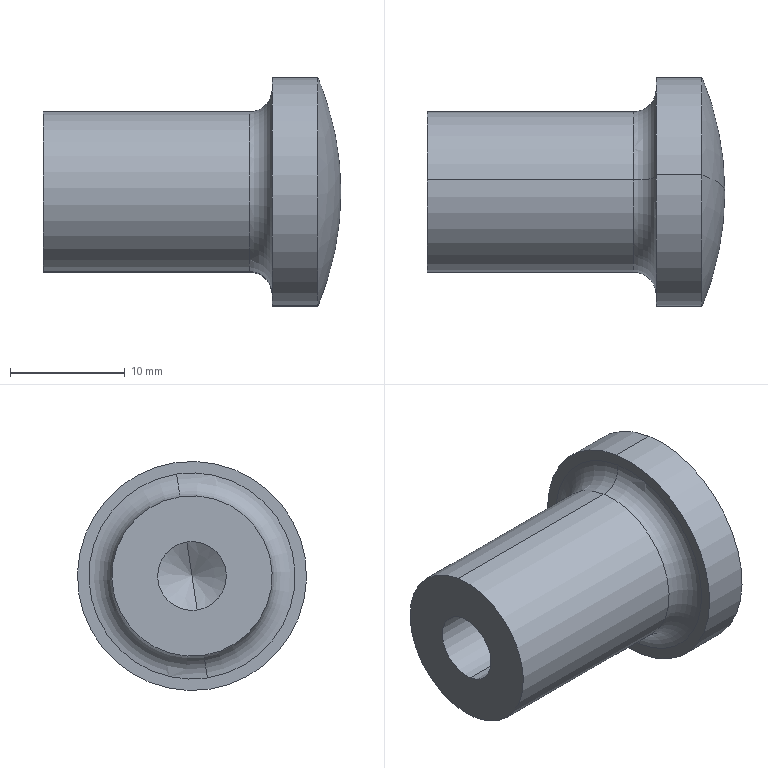Component | SolidWorks | STB-08-000-3-1_STB-08-027-1 | 1 solid | 14 faces | box 26 x 20 x 20 mm | volume 4196 mm3 | cylinder 6 | cone 2 | torus 2 | sphere 2 | plane 2 | commonest cylinder face diameters 6 x2 14 x2 20 x2
build123d program:
from build123d import *

# Parameters (mm, degrees)
SKETCH1_R             = 10
BOSS_EXTRUDE1_DEPTH   = 12
SKETCH2_OUTSIDE_W     = 29.418
SKETCH2_OUTSIDE_H     = 29.418
SKETCH2_OUTSIDE_R     = 7
CUT_EXTRUDE1_DEPTH    = 20
FILLET1_R             = 2
M6_TAPPED_HOLE1_D     = 6
M6_TAPPED_HOLE1_DEPTH = 17
M6_TAPPED_HOLE1_TIP   = 1.803
DOME1_FACE_RADIUS     = 10
DOME1_HEIGHT          = 2


with BuildPart() as part:
    # Sketch1 → Boss-Extrude1 (new, symmetric)
    with BuildSketch(Plane(origin=(0, 0, 0), x_dir=(0, 0, -1), z_dir=(1, 0, 0))):
        Circle(SKETCH1_R)
    extrude(amount=BOSS_EXTRUDE1_DEPTH, both=True)

    # Sketch2 outside → Cut-Extrude1 (cut)
    with BuildSketch(Plane.ZY.offset(12)):
        Rectangle(SKETCH2_OUTSIDE_W, SKETCH2_OUTSIDE_H)
        Circle(SKETCH2_OUTSIDE_R, mode=Mode.SUBTRACT)
    extrude(amount=-CUT_EXTRUDE1_DEPTH, mode=Mode.SUBTRACT)

    # Fillet1
    fillet1_edges = [part.edges().sort_by_distance(p)[0] for p in [
        (8, 0, -7),
    ]]
    fillet(fillet1_edges, radius=FILLET1_R)

    # M6 Tapped Hole1
    with Locations(Plane.ZY.offset(12)):
        with Locations((0, 0)):
            Hole(M6_TAPPED_HOLE1_D / 2, depth=M6_TAPPED_HOLE1_DEPTH)
            with Locations((0, 0, -(M6_TAPPED_HOLE1_DEPTH + M6_TAPPED_HOLE1_TIP / 2))):  # 118° drill point
                Cone(0, M6_TAPPED_HOLE1_D / 2, M6_TAPPED_HOLE1_TIP, mode=Mode.SUBTRACT)

    # Dome1: a dome of height H over a round flat face of radius A is a cap of a sphere of radius (A * A + H * H) / (2 * H)
    dome1_r = (DOME1_FACE_RADIUS * DOME1_FACE_RADIUS + DOME1_HEIGHT * DOME1_HEIGHT) / (2 * DOME1_HEIGHT)
    dome1_base = Plane((12, 0, 0), z_dir=(1, 0, 0))
    with Locations(dome1_base.offset(DOME1_HEIGHT - dome1_r)):
        dome1_ball = Sphere(dome1_r, mode=Mode.PRIVATE)
    add(split(dome1_ball, bisect_by=dome1_base, keep=Keep.TOP, mode=Mode.PRIVATE))


solid = part.part

# Placed as in the assembly
solid = solid.moved(Location((-207.904, 437.999, -10), (0, 0, 0)))
STEP:
#1=CARTESIAN_POINT('',(-7.988,17.226,-0.5105));
#2=VERTEX_POINT('',#1);
#3=CARTESIAN_POINT('',(-7.988,17.262,-0.2769));
#4=VERTEX_POINT('',#3);
#5=CARTESIAN_POINT('',(-7.988,17.244,-0.3937));
#6=DIRECTION('',(-1.,0.,0.));
#7=DIRECTION('',(0.,0.1487,0.9889));
#8=AXIS2_PLACEMENT_3D('',#5,#6,#7);
#9=CIRCLE('',#8,0.1181);
#10=EDGE_CURVE('',#2,#4,#9,.T.);
#11=ORIENTED_EDGE('',*,*,#10,.F.);
#12=CARTESIAN_POINT('',(-8.658,17.226,-0.5105));
#13=VERTEX_POINT('',#12);
#14=CARTESIAN_POINT('',(-8.658,17.226,-0.5105));
#15=DIRECTION('',(-1.,0.,0.));
#16=VECTOR('',#15,39.37);
#17=LINE('',#14,#16);
#18=EDGE_CURVE('',#2,#13,#17,.T.);
#19=ORIENTED_EDGE('',*,*,#18,.T.);
#20=CARTESIAN_POINT('',(-8.658,17.262,-0.2769));
#21=VERTEX_POINT('',#20);
#22=CARTESIAN_POINT('',(-8.658,17.244,-0.3937));
#23=DIRECTION('',(-1.,0.,0.));
#24=DIRECTION('',(0.,0.1487,0.9889));
#25=AXIS2_PLACEMENT_3D('',#22,#23,#24);
#26=CIRCLE('',#25,0.1181);
#27=EDGE_CURVE('',#13,#21,#26,.T.);
#28=ORIENTED_EDGE('',*,*,#27,.T.);
#29=CARTESIAN_POINT('',(-8.658,17.262,-0.2769));
#30=DIRECTION('',(-1.,0.,0.));
#31=VECTOR('',#30,39.37);
#32=LINE('',#29,#31);
#33=EDGE_CURVE('',#4,#21,#32,.T.);
#34=ORIENTED_EDGE('',*,*,#33,.F.);
#35=EDGE_LOOP('',(#11,#19,#28,#34));
#36=FACE_OUTER_BOUND('',#35,.T.);
#37=CARTESIAN_POINT('',(-8.658,17.244,-0.3937));
#38=DIRECTION('',(-1.,0.,0.));
#39=DIRECTION('',(0.,0.1487,0.9889));
#40=AXIS2_PLACEMENT_3D('',#37,#38,#39);
#41=CYLINDRICAL_SURFACE('',#40,0.1181);
#42=ADVANCED_FACE('',(#36),#41,.F.);
#43=CARTESIAN_POINT('',(-7.917,17.244,-0.3937));
#44=VERTEX_POINT('',#43);
#45=CARTESIAN_POINT('',(-7.988,17.262,-0.2769));
#46=DIRECTION('',(-0.515,0.1274,0.8476));
#47=VECTOR('',#46,39.37);
#48=LINE('',#45,#47);
#49=EDGE_CURVE('',#44,#4,#48,.T.);
#50=ORIENTED_EDGE('',*,*,#49,.F.);
#51=CARTESIAN_POINT('',(-7.988,17.226,-0.5105));
#52=DIRECTION('',(-0.515,-0.1274,-0.8476));
#53=VECTOR('',#52,39.37);
#54=LINE('',#51,#53);
#55=EDGE_CURVE('',#44,#2,#54,.T.);
#56=ORIENTED_EDGE('',*,*,#55,.T.);
#57=ORIENTED_EDGE('',*,*,#10,.T.);
#58=EDGE_LOOP('',(#50,#56,#57));
#59=FACE_OUTER_BOUND('',#58,.T.);
#60=CARTESIAN_POINT('',(-7.988,17.244,-0.3937));
#61=DIRECTION('',(-1.,0.,0.));
#62=DIRECTION('',(0.,0.1487,0.9889));
#63=AXIS2_PLACEMENT_3D('',#60,#61,#62);
#64=CONICAL_SURFACE('',#63,0.1181,1.03);
#65=ADVANCED_FACE('',(#59),#64,.F.);
#66=CARTESIAN_POINT('',(-7.949,17.203,-0.6662));
#67=VERTEX_POINT('',#66);
#68=CARTESIAN_POINT('',(-7.949,17.285,-0.1212));
#69=VERTEX_POINT('',#68);
#70=CARTESIAN_POINT('',(-7.949,17.244,-0.3937));
#71=DIRECTION('',(-1.,0.,0.));
#72=DIRECTION('',(0.,0.1487,0.9889));
#73=AXIS2_PLACEMENT_3D('',#70,#71,#72);
#74=CIRCLE('',#73,0.2756);
#75=EDGE_CURVE('',#67,#69,#74,.T.);
#76=ORIENTED_EDGE('',*,*,#75,.F.);
#77=CARTESIAN_POINT('',(-7.87,17.191,-0.7441));
#78=VERTEX_POINT('',#77);
#79=CARTESIAN_POINT('',(-7.949,17.191,-0.7441));
#80=DIRECTION('',(0.,0.9889,-0.1487));
#81=DIRECTION('',(0.,0.1487,0.9889));
#82=AXIS2_PLACEMENT_3D('',#79,#80,#81);
#83=CIRCLE('',#82,0.07874);
#84=EDGE_CURVE('',#67,#78,#83,.T.);
#85=ORIENTED_EDGE('',*,*,#84,.T.);
#86=CARTESIAN_POINT('',(-7.87,17.297,-0.04331));
#87=VERTEX_POINT('',#86);
#88=CARTESIAN_POINT('',(-7.87,17.244,-0.3937));
#89=DIRECTION('',(1.,0.,0.));
#90=DIRECTION('',(0.,0.1487,0.9889));
#91=AXIS2_PLACEMENT_3D('',#88,#89,#90);
#92=CIRCLE('',#91,0.3543);
#93=EDGE_CURVE('',#87,#78,#92,.T.);
#94=ORIENTED_EDGE('',*,*,#93,.F.);
#95=CARTESIAN_POINT('',(-7.949,17.297,-0.04331));
#96=DIRECTION('',(0.,-0.9889,0.1487));
#97=DIRECTION('',(0.,-0.1487,-0.9889));
#98=AXIS2_PLACEMENT_3D('',#95,#96,#97);
#99=CIRCLE('',#98,0.07874);
#100=EDGE_CURVE('',#69,#87,#99,.T.);
#101=ORIENTED_EDGE('',*,*,#100,.F.);
#102=EDGE_LOOP('',(#76,#85,#94,#101));
#103=FACE_OUTER_BOUND('',#102,.T.);
#104=CARTESIAN_POINT('',(-7.949,17.244,-0.3937));
#105=DIRECTION('',(-1.,0.,0.));
#106=DIRECTION('',(0.,0.1487,0.9889));
#107=AXIS2_PLACEMENT_3D('',#104,#105,#106);
#108=TOROIDAL_SURFACE('',#107,0.3543,0.07874);
#109=ADVANCED_FACE('',(#103),#108,.F.);
#110=CARTESIAN_POINT('',(-7.949,17.244,-0.3937));
#111=DIRECTION('',(-1.,0.,0.));
#112=DIRECTION('',(0.,0.1487,0.9889));
#113=AXIS2_PLACEMENT_3D('',#110,#111,#112);
#114=CIRCLE('',#113,0.2756);
#115=EDGE_CURVE('',#69,#67,#114,.T.);
#116=ORIENTED_EDGE('',*,*,#115,.T.);
#117=CARTESIAN_POINT('',(-8.658,17.203,-0.6662));
#118=VERTEX_POINT('',#117);
#119=CARTESIAN_POINT('',(-7.87,17.203,-0.6662));
#120=DIRECTION('',(-1.,0.,0.));
#121=VECTOR('',#120,39.37);
#122=LINE('',#119,#121);
#123=EDGE_CURVE('',#67,#118,#122,.T.);
#124=ORIENTED_EDGE('',*,*,#123,.T.);
#125=CARTESIAN_POINT('',(-8.658,17.285,-0.1212));
#126=VERTEX_POINT('',#125);
#127=CARTESIAN_POINT('',(-8.658,17.244,-0.3937));
#128=DIRECTION('',(-1.,0.,0.));
#129=DIRECTION('',(0.,0.1487,0.9889));
#130=AXIS2_PLACEMENT_3D('',#127,#128,#129);
#131=CIRCLE('',#130,0.2756);
#132=EDGE_CURVE('',#126,#118,#131,.T.);
#133=ORIENTED_EDGE('',*,*,#132,.F.);
#134=CARTESIAN_POINT('',(-7.87,17.285,-0.1212));
#135=DIRECTION('',(-1.,0.,0.));
#136=VECTOR('',#135,39.37);
#137=LINE('',#134,#136);
#138=EDGE_CURVE('',#69,#126,#137,.T.);
#139=ORIENTED_EDGE('',*,*,#138,.F.);
#140=EDGE_LOOP('',(#116,#124,#133,#139));
#141=FACE_OUTER_BOUND('',#140,.T.);
#142=CARTESIAN_POINT('',(-7.87,17.244,-0.3937));
#143=DIRECTION('',(-1.,0.,0.));
#144=DIRECTION('',(0.,0.1487,0.9889));
#145=AXIS2_PLACEMENT_3D('',#142,#143,#144);
#146=CYLINDRICAL_SURFACE('',#145,0.2756);
#147=ADVANCED_FACE('',(#141),#146,.T.);
#148=CARTESIAN_POINT('',(-7.713,17.303,-0.004375));
#149=VERTEX_POINT('',#148);
#150=CARTESIAN_POINT('',(-7.713,17.186,-0.783));
#151=VERTEX_POINT('',#150);
#152=CARTESIAN_POINT('',(-7.713,17.244,-0.3937));
#153=DIRECTION('',(1.,0.,0.));
#154=DIRECTION('',(0.,-0.1487,-0.9889));
#155=AXIS2_PLACEMENT_3D('',#152,#153,#154);
#156=CIRCLE('',#155,0.3937);
#157=EDGE_CURVE('',#149,#151,#156,.T.);
#158=ORIENTED_EDGE('',*,*,#157,.T.);
#159=CARTESIAN_POINT('',(-8.658,17.244,-0.3937));
#160=DIRECTION('',(0.,-0.9889,0.1487));
#161=DIRECTION('',(0.,-0.1487,-0.9889));
#162=AXIS2_PLACEMENT_3D('',#159,#160,#161);
#163=CIRCLE('',#162,1.024);
#164=EDGE_CURVE('',#151,#149,#163,.T.);
#165=ORIENTED_EDGE('',*,*,#164,.T.);
#166=EDGE_LOOP('',(#158,#165));
#167=FACE_OUTER_BOUND('',#166,.T.);
#168=CARTESIAN_POINT('',(-8.658,17.244,-0.3937));
#169=DIRECTION('',(0.,0.9889,-0.1487));
#170=DIRECTION('',(1.,0.,0.));
#171=AXIS2_PLACEMENT_3D('',#168,#169,#170);
#172=SPHERICAL_SURFACE('',#171,1.024);
#173=ADVANCED_FACE('',(#167),#172,.T.);
#174=CARTESIAN_POINT('',(-7.713,17.244,-0.3937));
#175=DIRECTION('',(1.,0.,0.));
#176=DIRECTION('',(0.,-0.1487,-0.9889));
#177=AXIS2_PLACEMENT_3D('',#174,#175,#176);
#178=CIRCLE('',#177,0.3937);
#179=EDGE_CURVE('',#151,#149,#178,.T.);
#180=ORIENTED_EDGE('',*,*,#179,.F.);
#181=CARTESIAN_POINT('',(-7.87,17.186,-0.783));
#182=VERTEX_POINT('',#181);
#183=CARTESIAN_POINT('',(-7.713,17.186,-0.783));
#184=DIRECTION('',(-1.,0.,0.));
#185=VECTOR('',#184,39.37);
#186=LINE('',#183,#185);
#187=EDGE_CURVE('',#151,#182,#186,.T.);
#188=ORIENTED_EDGE('',*,*,#187,.T.);
#189=CARTESIAN_POINT('',(-7.87,17.303,-0.004375));
#190=VERTEX_POINT('',#189);
#191=CARTESIAN_POINT('',(-7.87,17.244,-0.3937));
#192=DIRECTION('',(-1.,0.,0.));
#193=DIRECTION('',(0.,0.1487,0.9889));
#194=AXIS2_PLACEMENT_3D('',#191,#192,#193);
#195=CIRCLE('',#194,0.3937);
#196=EDGE_CURVE('',#190,#182,#195,.T.);
#197=ORIENTED_EDGE('',*,*,#196,.F.);
#198=CARTESIAN_POINT('',(-7.713,17.303,-0.004375));
#199=DIRECTION('',(-1.,0.,0.));
#200=VECTOR('',#199,39.37);
#201=LINE('',#198,#200);
#202=EDGE_CURVE('',#149,#190,#201,.T.);
#203=ORIENTED_EDGE('',*,*,#202,.F.);
#204=EDGE_LOOP('',(#180,#188,#197,#203));
#205=FACE_OUTER_BOUND('',#204,.T.);
#206=CARTESIAN_POINT('',(-7.713,17.244,-0.3937));
#207=DIRECTION('',(-1.,0.,0.));
#208=DIRECTION('',(0.,0.1487,0.9889));
#209=AXIS2_PLACEMENT_3D('',#206,#207,#208);
#210=CYLINDRICAL_SURFACE('',#209,0.3937);
#211=ADVANCED_FACE('',(#205),#210,.T.);
#212=ORIENTED_EDGE('',*,*,#187,.F.);
#213=ORIENTED_EDGE('',*,*,#157,.F.);
#214=ORIENTED_EDGE('',*,*,#202,.T.);
#215=CARTESIAN_POINT('',(-7.87,17.244,-0.3937));
#216=DIRECTION('',(-1.,0.,0.));
#217=DIRECTION('',(0.,0.1487,0.9889));
#218=AXIS2_PLACEMENT_3D('',#215,#216,#217);
#219=CIRCLE('',#218,0.3937);
#220=EDGE_CURVE('',#182,#190,#219,.T.);
#221=ORIENTED_EDGE('',*,*,#220,.F.);
#222=EDGE_LOOP('',(#212,#213,#214,#221));
#223=FACE_OUTER_BOUND('',#222,.T.);
#224=CARTESIAN_POINT('',(-7.713,17.244,-0.3937));
#225=DIRECTION('',(-1.,0.,0.));
#226=DIRECTION('',(0.,0.1487,0.9889));
#227=AXIS2_PLACEMENT_3D('',#224,#225,#226);
#228=CYLINDRICAL_SURFACE('',#227,0.3937);
#229=ADVANCED_FACE('',(#223),#228,.T.);
#230=ORIENTED_EDGE('',*,*,#164,.F.);
#231=ORIENTED_EDGE('',*,*,#179,.T.);
#232=EDGE_LOOP('',(#230,#231));
#233=FACE_OUTER_BOUND('',#232,.T.);
#234=CARTESIAN_POINT('',(-8.658,17.244,-0.3937));
#235=DIRECTION('',(0.,0.9889,-0.1487));
#236=DIRECTION('',(1.,0.,0.));
#237=AXIS2_PLACEMENT_3D('',#234,#235,#236);
#238=SPHERICAL_SURFACE('',#237,1.024);
#239=ADVANCED_FACE('',(#233),#238,.T.);
#240=ORIENTED_EDGE('',*,*,#93,.T.);
#241=CARTESIAN_POINT('',(-7.87,17.244,-0.3937));
#242=DIRECTION('',(1.,0.,0.));
#243=DIRECTION('',(0.,0.1487,0.9889));
#244=AXIS2_PLACEMENT_3D('',#241,#242,#243);
#245=CIRCLE('',#244,0.3543);
#246=EDGE_CURVE('',#78,#87,#245,.T.);
#247=ORIENTED_EDGE('',*,*,#246,.T.);
#248=EDGE_LOOP('',(#240,#247));
#249=FACE_BOUND('',#248,.T.);
#250=ORIENTED_EDGE('',*,*,#196,.T.);
#251=ORIENTED_EDGE('',*,*,#220,.T.);
#252=EDGE_LOOP('',(#250,#251));
#253=FACE_OUTER_BOUND('',#252,.T.);
#254=CARTESIAN_POINT('',(-7.87,17.244,-0.3937));
#255=DIRECTION('',(-1.,0.,0.));
#256=DIRECTION('',(0.,0.1487,0.9889));
#257=AXIS2_PLACEMENT_3D('',#254,#255,#256);
#258=PLANE('',#257);
#259=ADVANCED_FACE('',(#249,#253),#258,.T.);
#260=ORIENTED_EDGE('',*,*,#123,.F.);
#261=ORIENTED_EDGE('',*,*,#75,.T.);
#262=ORIENTED_EDGE('',*,*,#138,.T.);
#263=CARTESIAN_POINT('',(-8.658,17.244,-0.3937));
#264=DIRECTION('',(-1.,0.,0.));
#265=DIRECTION('',(0.,0.1487,0.9889));
#266=AXIS2_PLACEMENT_3D('',#263,#264,#265);
#267=CIRCLE('',#266,0.2756);
#268=EDGE_CURVE('',#118,#126,#267,.T.);
#269=ORIENTED_EDGE('',*,*,#268,.F.);
#270=EDGE_LOOP('',(#260,#261,#262,#269));
#271=FACE_OUTER_BOUND('',#270,.T.);
#272=CARTESIAN_POINT('',(-7.87,17.244,-0.3937));
#273=DIRECTION('',(-1.,0.,0.));
#274=DIRECTION('',(0.,0.1487,0.9889));
#275=AXIS2_PLACEMENT_3D('',#272,#273,#274);
#276=CYLINDRICAL_SURFACE('',#275,0.2756);
#277=ADVANCED_FACE('',(#271),#276,.T.);
#278=CARTESIAN_POINT('',(-8.658,17.244,-0.3937));
#279=DIRECTION('',(-1.,0.,0.));
#280=DIRECTION('',(0.,0.1487,0.9889));
#281=AXIS2_PLACEMENT_3D('',#278,#279,#280);
#282=CIRCLE('',#281,0.1181);
#283=EDGE_CURVE('',#21,#13,#282,.T.);
#284=ORIENTED_EDGE('',*,*,#283,.F.);
#285=ORIENTED_EDGE('',*,*,#27,.F.);
#286=EDGE_LOOP('',(#284,#285));
#287=FACE_BOUND('',#286,.T.);
#288=ORIENTED_EDGE('',*,*,#132,.T.);
#289=ORIENTED_EDGE('',*,*,#268,.T.);
#290=EDGE_LOOP('',(#288,#289));
#291=FACE_OUTER_BOUND('',#290,.T.);
#292=CARTESIAN_POINT('',(-8.658,17.244,-0.3937));
#293=DIRECTION('',(1.,0.,0.));
#294=DIRECTION('',(0.,-0.1487,-0.9889));
#295=AXIS2_PLACEMENT_3D('',#292,#293,#294);
#296=PLANE('',#295);
#297=ADVANCED_FACE('',(#287,#291),#296,.F.);
#298=ORIENTED_EDGE('',*,*,#84,.F.);
#299=ORIENTED_EDGE('',*,*,#115,.F.);
#300=ORIENTED_EDGE('',*,*,#100,.T.);
#301=ORIENTED_EDGE('',*,*,#246,.F.);
#302=EDGE_LOOP('',(#298,#299,#300,#301));
#303=FACE_OUTER_BOUND('',#302,.T.);
#304=CARTESIAN_POINT('',(-7.949,17.244,-0.3937));
#305=DIRECTION('',(-1.,0.,0.));
#306=DIRECTION('',(0.,0.1487,0.9889));
#307=AXIS2_PLACEMENT_3D('',#304,#305,#306);
#308=TOROIDAL_SURFACE('',#307,0.3543,0.07874);
#309=ADVANCED_FACE('',(#303),#308,.F.);
#310=ORIENTED_EDGE('',*,*,#55,.F.);
#311=ORIENTED_EDGE('',*,*,#49,.T.);
#312=CARTESIAN_POINT('',(-7.988,17.244,-0.3937));
#313=DIRECTION('',(-1.,0.,0.));
#314=DIRECTION('',(0.,0.1487,0.9889));
#315=AXIS2_PLACEMENT_3D('',#312,#313,#314);
#316=CIRCLE('',#315,0.1181);
#317=EDGE_CURVE('',#4,#2,#316,.T.);
#318=ORIENTED_EDGE('',*,*,#317,.T.);
#319=EDGE_LOOP('',(#310,#311,#318));
#320=FACE_OUTER_BOUND('',#319,.T.);
#321=CARTESIAN_POINT('',(-7.988,17.244,-0.3937));
#322=DIRECTION('',(-1.,0.,0.));
#323=DIRECTION('',(0.,0.1487,0.9889));
#324=AXIS2_PLACEMENT_3D('',#321,#322,#323);
#325=CONICAL_SURFACE('',#324,0.1181,1.03);
#326=ADVANCED_FACE('',(#320),#325,.F.);
#327=ORIENTED_EDGE('',*,*,#18,.F.);
#328=ORIENTED_EDGE('',*,*,#317,.F.);
#329=ORIENTED_EDGE('',*,*,#33,.T.);
#330=ORIENTED_EDGE('',*,*,#283,.T.);
#331=EDGE_LOOP('',(#327,#328,#329,#330));
#332=FACE_OUTER_BOUND('',#331,.T.);
#333=CARTESIAN_POINT('',(-8.658,17.244,-0.3937));
#334=DIRECTION('',(-1.,0.,0.));
#335=DIRECTION('',(0.,0.1487,0.9889));
#336=AXIS2_PLACEMENT_3D('',#333,#334,#335);
#337=CYLINDRICAL_SURFACE('',#336,0.1181);
#338=ADVANCED_FACE('',(#332),#337,.F.);
#339=CLOSED_SHELL('',(#42,#65,#109,#147,#173,#211,#229,#239,#259,#277,#297,#309,#326,#338));
#340=MANIFOLD_SOLID_BREP('',#339);
#341=CARTESIAN_POINT('',(0.,0.,0.));
#342=DIRECTION('',(0.,0.,1.));
#343=DIRECTION('',(1.,0.,0.));
#344=AXIS2_PLACEMENT_3D('',#341,#342,#343);
#345=(LENGTH_UNIT()NAMED_UNIT(*)SI_UNIT($,.METRE.));
#346=LENGTH_MEASURE_WITH_UNIT(LENGTH_MEASURE(0.0254),#345);
#347=DIMENSIONAL_EXPONENTS(1.,0.,0.,0.,0.,0.,0.);
#348=(CONVERSION_BASED_UNIT('',#346)LENGTH_UNIT()NAMED_UNIT(#347));
#349=UNCERTAINTY_MEASURE_WITH_UNIT(LENGTH_MEASURE(0.00001),#348,'','');
#350=(NAMED_UNIT(*)PLANE_ANGLE_UNIT()SI_UNIT($,.RADIAN.));
#351=(NAMED_UNIT(*)SI_UNIT($,.STERADIAN.)SOLID_ANGLE_UNIT());
#352=(GEOMETRIC_REPRESENTATION_CONTEXT(3)GLOBAL_UNCERTAINTY_ASSIGNED_CONTEXT((#349))GLOBAL_UNIT_ASSIGNED_CONTEXT((#348,#350,#351))REPRESENTATION_CONTEXT('',''));
#353=ADVANCED_BREP_SHAPE_REPRESENTATION('',(#340,#344),#352);
#354=COLOUR_RGB('',0.7922,0.8196,0.9333);
#355=FILL_AREA_STYLE_COLOUR('',#354);
#356=FILL_AREA_STYLE('',(#355));
#357=SURFACE_STYLE_FILL_AREA(#356);
#358=SURFACE_SIDE_STYLE('',(#357));
#359=SURFACE_STYLE_USAGE(.BOTH.,#358);
#360=PRESENTATION_STYLE_ASSIGNMENT((#359));
#361=STYLED_ITEM('',(#360),#340);
#362=(LENGTH_UNIT()NAMED_UNIT(*)SI_UNIT($,.METRE.));
#363=LENGTH_MEASURE_WITH_UNIT(LENGTH_MEASURE(0.0254),#362);
#364=DIMENSIONAL_EXPONENTS(1.,0.,0.,0.,0.,0.,0.);
#365=(CONVERSION_BASED_UNIT('',#363)LENGTH_UNIT()NAMED_UNIT(#364));
#366=UNCERTAINTY_MEASURE_WITH_UNIT(LENGTH_MEASURE(0.00001),#365,'','');
#367=(NAMED_UNIT(*)PLANE_ANGLE_UNIT()SI_UNIT($,.RADIAN.));
#368=(NAMED_UNIT(*)SI_UNIT($,.STERADIAN.)SOLID_ANGLE_UNIT());
#369=(GEOMETRIC_REPRESENTATION_CONTEXT(3)GLOBAL_UNCERTAINTY_ASSIGNED_CONTEXT((#366))GLOBAL_UNIT_ASSIGNED_CONTEXT((#365,#367,#368))REPRESENTATION_CONTEXT('',''));
#370=MECHANICAL_DESIGN_GEOMETRIC_PRESENTATION_REPRESENTATION('',(#361),#369);
#371=PRESENTATION_LAYER_ASSIGNMENT('','',(#361));